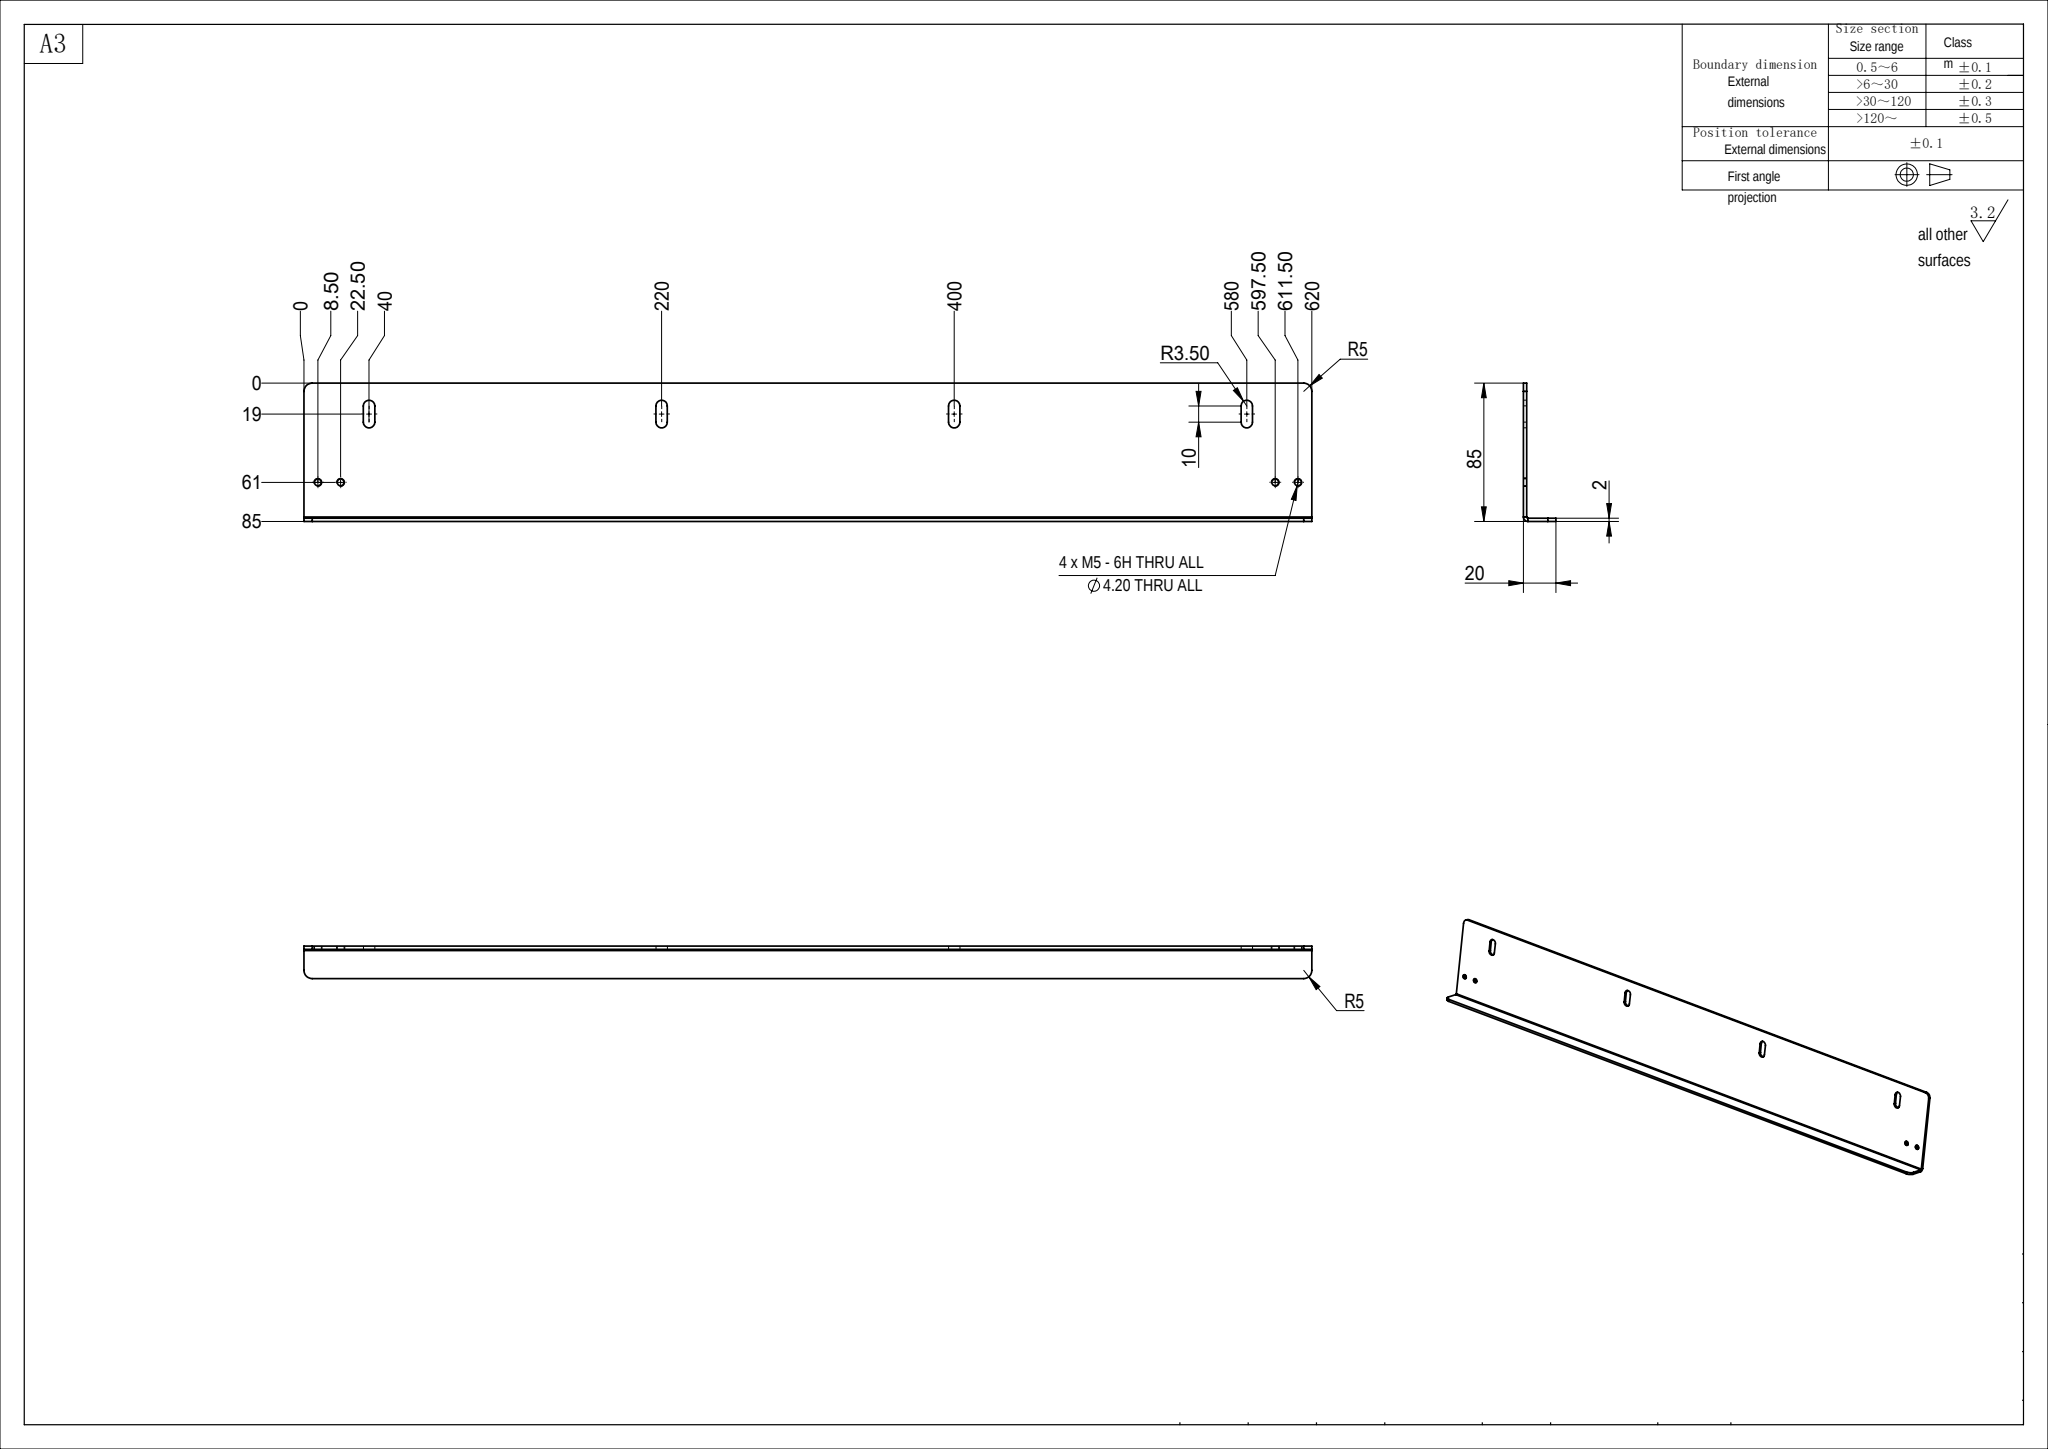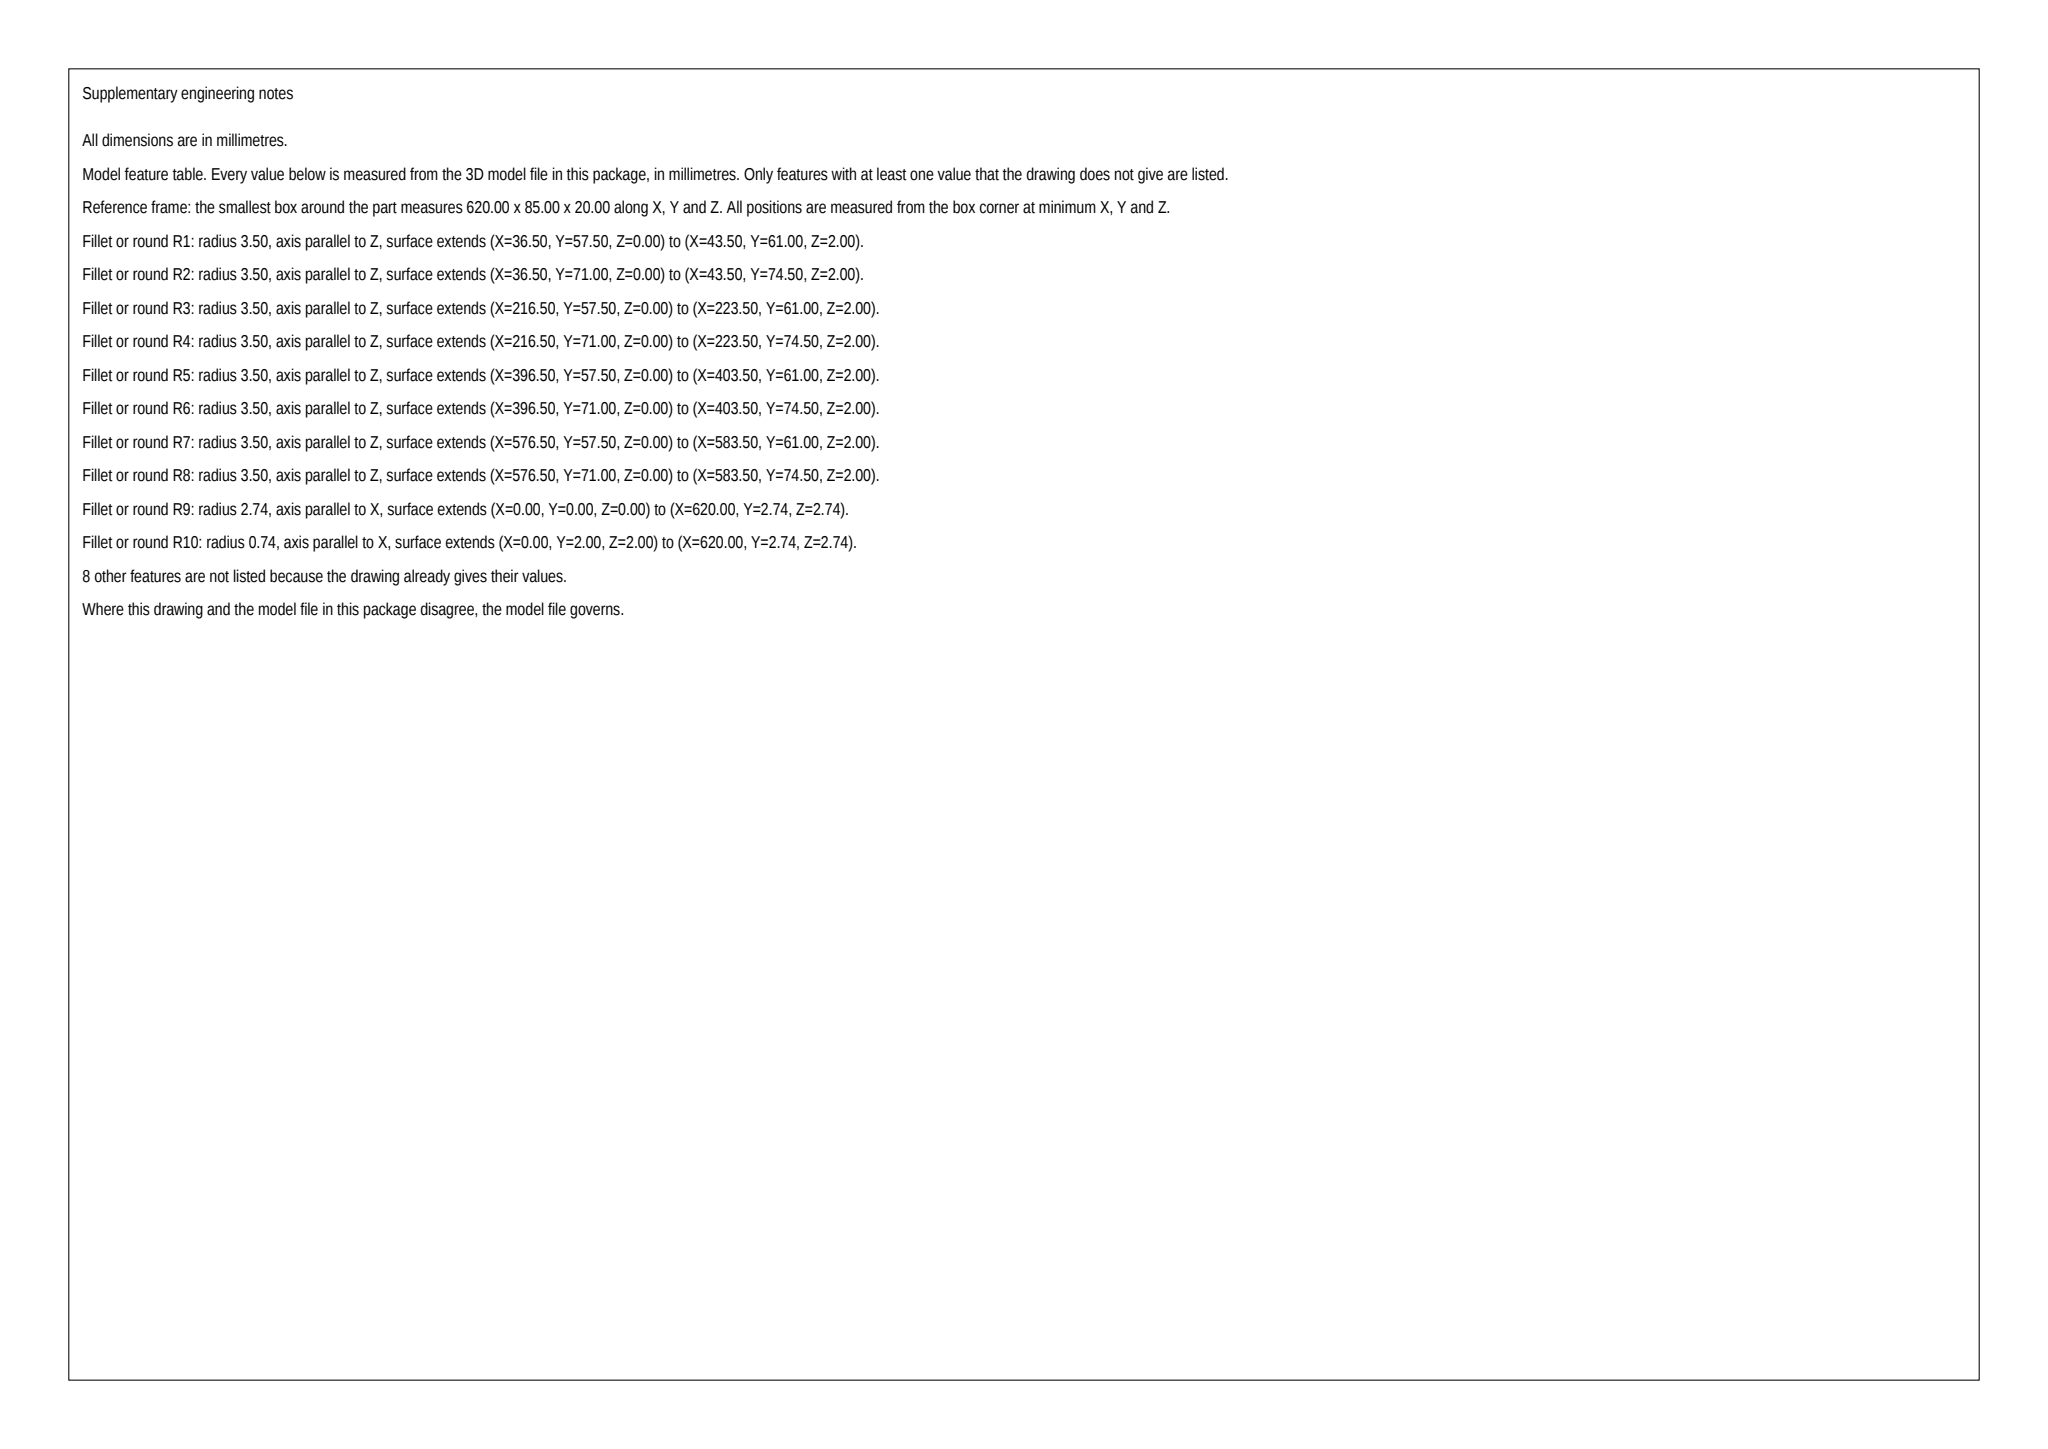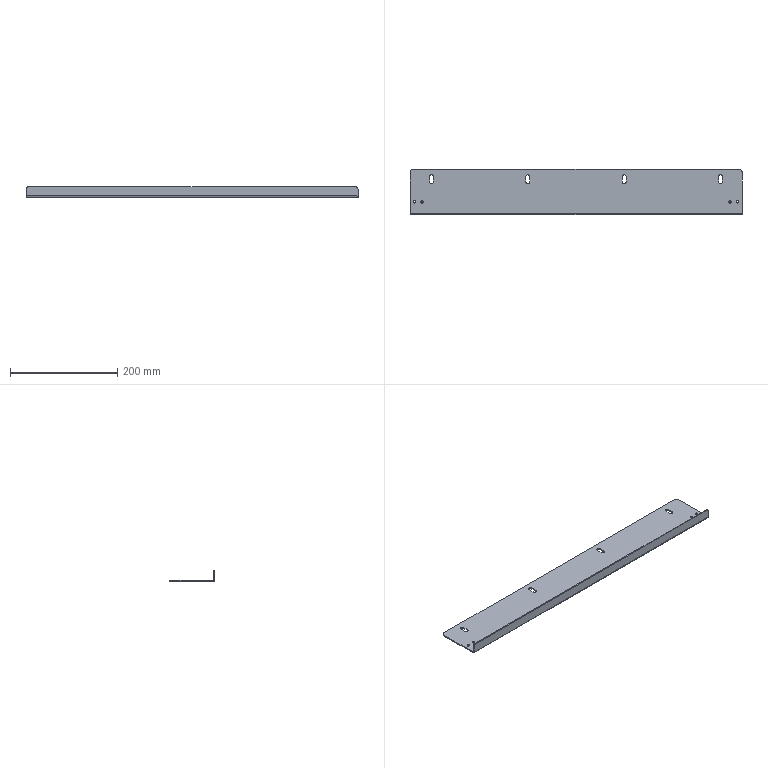Part | SolidWorks | mm | 1 solid | 42 faces | box 620 x 85 x 20 mm | volume 125774 mm3 | cylinder 22 | plane 20 | commonest cylinder face diameters 4.2 x8 7 x8 10 x4 5.473 x1 1.473 x1